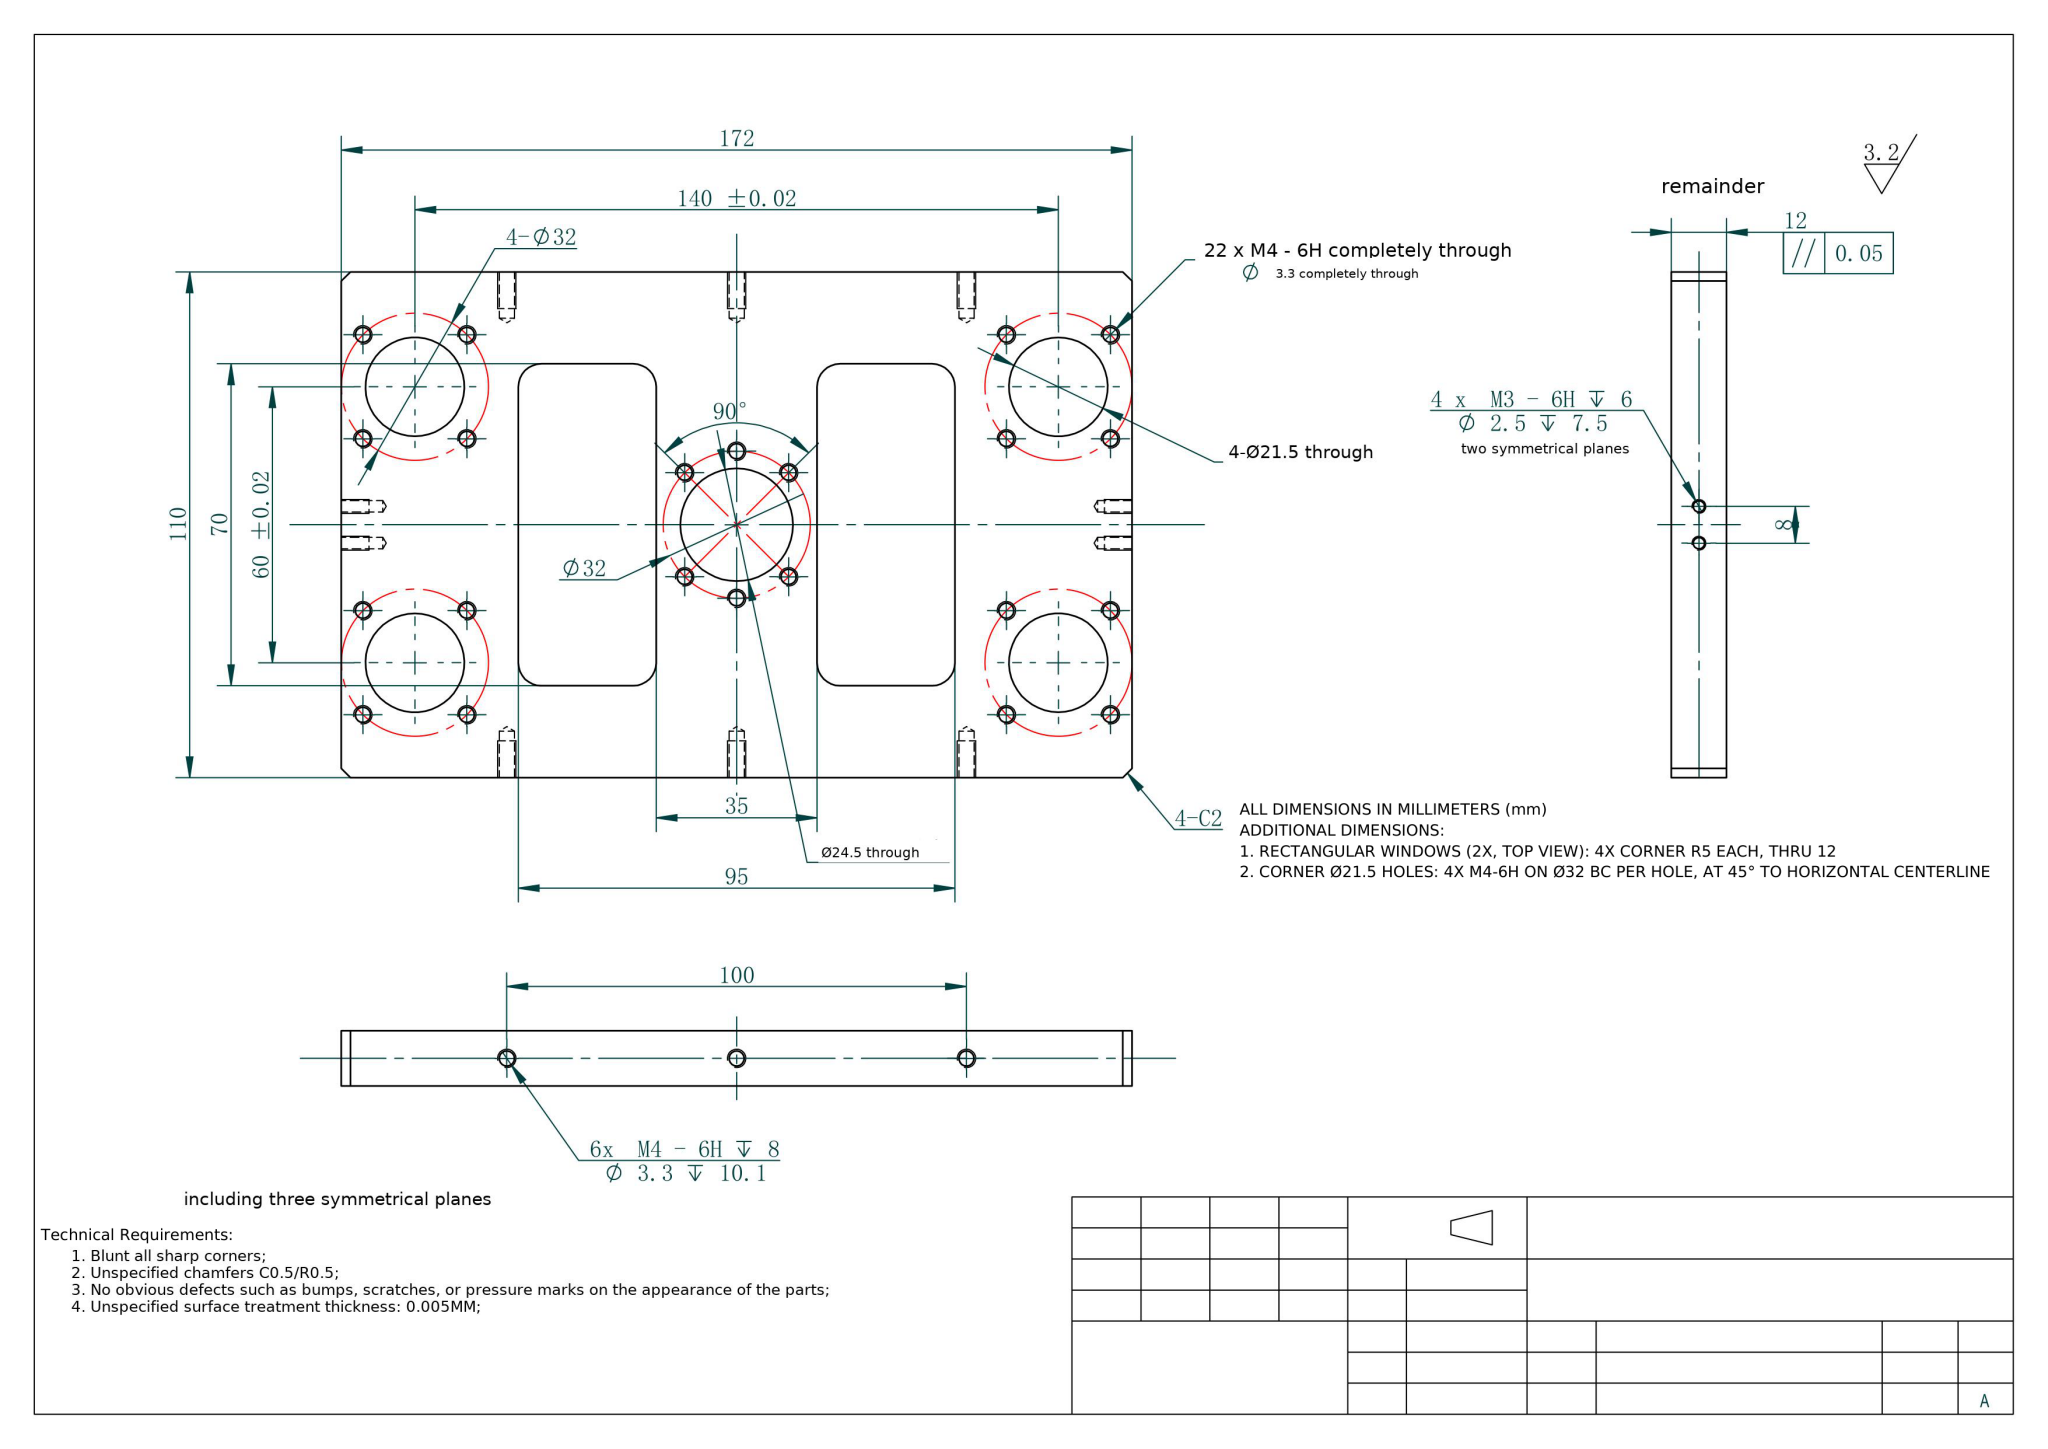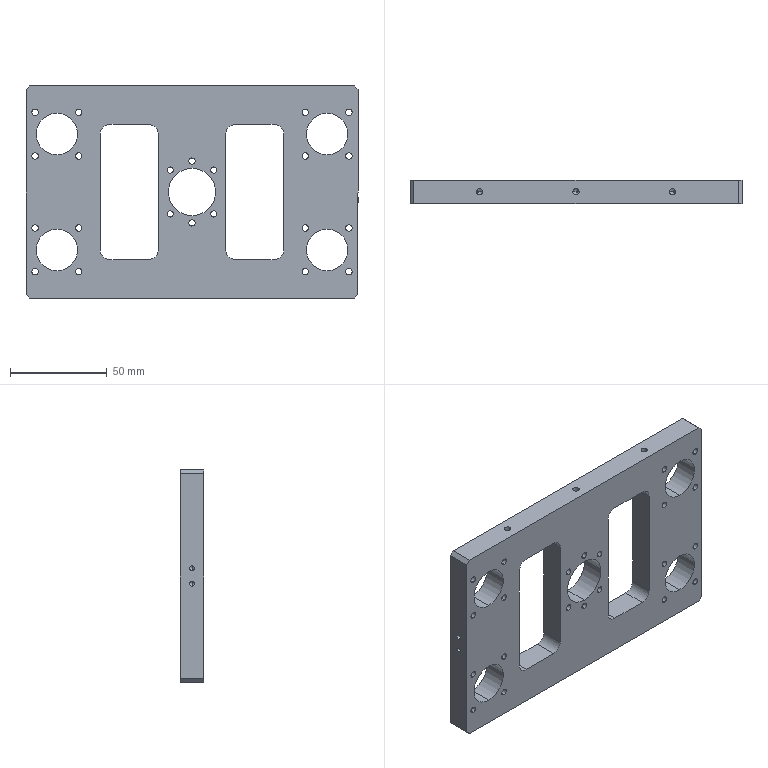Part | NX | mm | 1 solid | 120 faces | box 172 x 12 x 110 mm | volume 151015 mm3 | cylinder 82 | cone 20 | plane 18 | commonest cylinder face diameters 3.3 x56 2.5 x8 21.5 x8 10 x8 24.5 x2